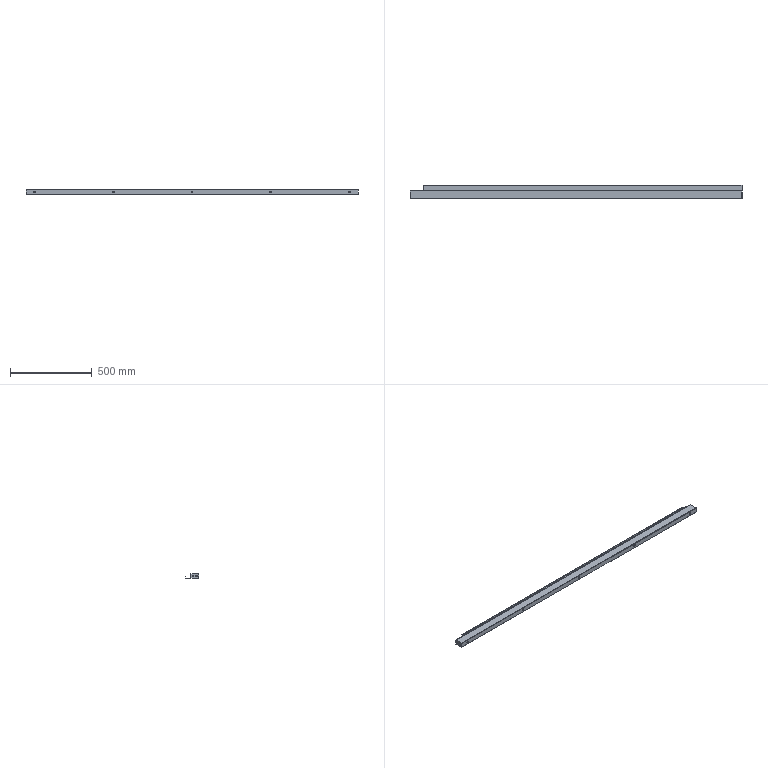Component | SolidWorks | LowerCrossbeam1234-1 | 1 solid | 80 faces | volume 444825 mm3 | plane 50 | cylinder 30 | commonest cylinder face diameters 11 x14 3.4 x6 0.4 x6 9 x4